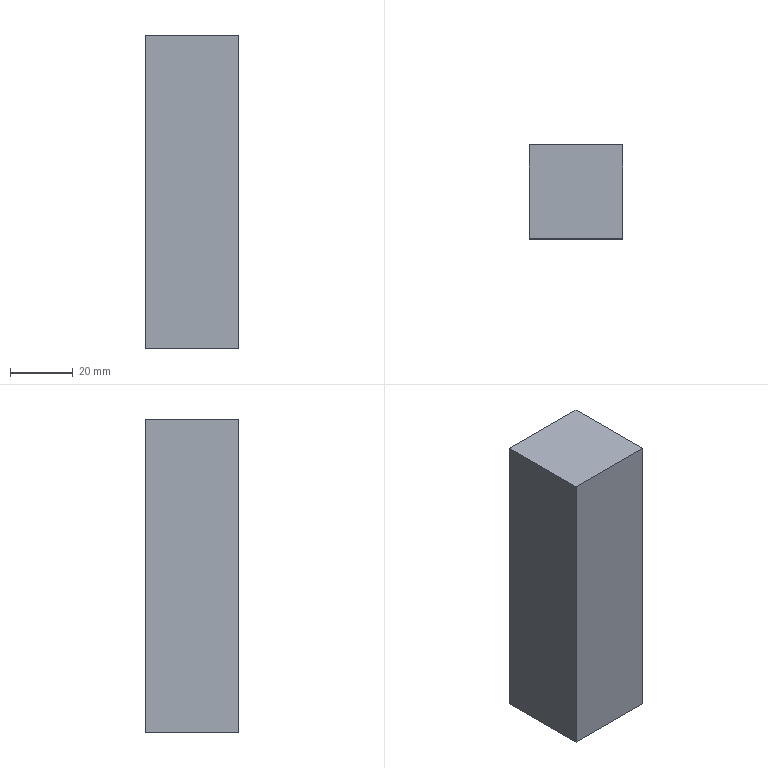Component | NX | FRONT_UP | 1 solid | 6 faces | box 30 x 30 x 100 mm | volume 90000 mm3 | plane 6
STEP:
#1=CARTESIAN_POINT('',(0.,0.,0.));
#2=DIRECTION('',(0.,0.,1.));
#3=DIRECTION('',(1.,0.,0.));
#4=AXIS2_PLACEMENT_3D('',#1,#2,#3);
#5=CARTESIAN_POINT('',(422.662,-30.,80.));
#6=VERTEX_POINT('',#5);
#7=CARTESIAN_POINT('',(422.662,-30.,-20.));
#8=VERTEX_POINT('',#7);
#9=CARTESIAN_POINT('',(422.662,-30.,80.));
#10=DIRECTION('',(0.,0.,-1.));
#11=VECTOR('',#10,1.);
#12=LINE('',#9,#11);
#13=CARTESIAN_POINT('',(422.662,-60.,80.));
#14=DIRECTION('',(1.,0.,0.));
#15=DIRECTION('',(0.,0.,-1.));
#16=AXIS2_PLACEMENT_3D('',#13,#14,#15);
#17=PLANE('',#16);
#18=CARTESIAN_POINT('',(0.,30.));
#19=DIRECTION('',(1.,0.));
#20=VECTOR('',#19,1.);
#21=LINE('',#18,#20);
#22=(GEOMETRIC_REPRESENTATION_CONTEXT(2)PARAMETRIC_REPRESENTATION_CONTEXT()REPRESENTATION_CONTEXT('',''));
#23=DEFINITIONAL_REPRESENTATION('',(#21),#22);
#24=PCURVE('',#17,#23);
#25=CARTESIAN_POINT('',(422.662,-30.,-20.));
#26=DIRECTION('',(0.,-1.,0.));
#27=DIRECTION('',(0.,0.,-1.));
#28=AXIS2_PLACEMENT_3D('',#25,#26,#27);
#29=PLANE('',#28);
#30=CARTESIAN_POINT('',(-100.,0.));
#31=DIRECTION('',(1.,0.));
#32=VECTOR('',#31,1.);
#33=LINE('',#30,#32);
#34=(GEOMETRIC_REPRESENTATION_CONTEXT(2)PARAMETRIC_REPRESENTATION_CONTEXT()REPRESENTATION_CONTEXT('',''));
#35=DEFINITIONAL_REPRESENTATION('',(#33),#34);
#36=PCURVE('',#29,#35);
#37=SURFACE_CURVE('',#12,(#24,#36),.PCURVE_S1.);
#38=EDGE_CURVE('',#6,#8,#37,.T.);
#39=ORIENTED_EDGE('',*,*,#38,.T.);
#40=CARTESIAN_POINT('',(422.662,-60.,-20.));
#41=VERTEX_POINT('',#40);
#42=CARTESIAN_POINT('',(422.662,-60.,-20.));
#43=DIRECTION('',(0.,1.,0.));
#44=VECTOR('',#43,1.);
#45=LINE('',#42,#44);
#46=CARTESIAN_POINT('',(100.,0.));
#47=DIRECTION('',(0.,1.));
#48=VECTOR('',#47,1.);
#49=LINE('',#46,#48);
#50=(GEOMETRIC_REPRESENTATION_CONTEXT(2)PARAMETRIC_REPRESENTATION_CONTEXT()REPRESENTATION_CONTEXT('',''));
#51=DEFINITIONAL_REPRESENTATION('',(#49),#50);
#52=PCURVE('',#17,#51);
#53=CARTESIAN_POINT('',(422.662,-60.,-20.));
#54=DIRECTION('',(0.,0.,1.));
#55=DIRECTION('',(1.,0.,0.));
#56=AXIS2_PLACEMENT_3D('',#53,#54,#55);
#57=PLANE('',#56);
#58=CARTESIAN_POINT('',(0.,0.));
#59=DIRECTION('',(0.,1.));
#60=VECTOR('',#59,1.);
#61=LINE('',#58,#60);
#62=(GEOMETRIC_REPRESENTATION_CONTEXT(2)PARAMETRIC_REPRESENTATION_CONTEXT()REPRESENTATION_CONTEXT('',''));
#63=DEFINITIONAL_REPRESENTATION('',(#61),#62);
#64=PCURVE('',#57,#63);
#65=SURFACE_CURVE('',#45,(#52,#64),.PCURVE_S1.);
#66=EDGE_CURVE('',#41,#8,#65,.T.);
#67=ORIENTED_EDGE('',*,*,#66,.F.);
#68=CARTESIAN_POINT('',(422.662,-60.,80.));
#69=VERTEX_POINT('',#68);
#70=CARTESIAN_POINT('',(422.662,-60.,80.));
#71=DIRECTION('',(0.,0.,-1.));
#72=VECTOR('',#71,1.);
#73=LINE('',#70,#72);
#74=CARTESIAN_POINT('',(0.,0.));
#75=DIRECTION('',(1.,0.));
#76=VECTOR('',#75,1.);
#77=LINE('',#74,#76);
#78=(GEOMETRIC_REPRESENTATION_CONTEXT(2)PARAMETRIC_REPRESENTATION_CONTEXT()REPRESENTATION_CONTEXT('',''));
#79=DEFINITIONAL_REPRESENTATION('',(#77),#78);
#80=PCURVE('',#17,#79);
#81=CARTESIAN_POINT('',(422.662,-60.,-20.));
#82=DIRECTION('',(0.,-1.,0.));
#83=DIRECTION('',(0.,0.,-1.));
#84=AXIS2_PLACEMENT_3D('',#81,#82,#83);
#85=PLANE('',#84);
#86=CARTESIAN_POINT('',(-100.,0.));
#87=DIRECTION('',(1.,0.));
#88=VECTOR('',#87,1.);
#89=LINE('',#86,#88);
#90=(GEOMETRIC_REPRESENTATION_CONTEXT(2)PARAMETRIC_REPRESENTATION_CONTEXT()REPRESENTATION_CONTEXT('',''));
#91=DEFINITIONAL_REPRESENTATION('',(#89),#90);
#92=PCURVE('',#85,#91);
#93=SURFACE_CURVE('',#73,(#80,#92),.PCURVE_S1.);
#94=EDGE_CURVE('',#69,#41,#93,.T.);
#95=ORIENTED_EDGE('',*,*,#94,.F.);
#96=CARTESIAN_POINT('',(422.662,-60.,80.));
#97=DIRECTION('',(0.,1.,0.));
#98=VECTOR('',#97,1.);
#99=LINE('',#96,#98);
#100=CARTESIAN_POINT('',(0.,0.));
#101=DIRECTION('',(0.,1.));
#102=VECTOR('',#101,1.);
#103=LINE('',#100,#102);
#104=(GEOMETRIC_REPRESENTATION_CONTEXT(2)PARAMETRIC_REPRESENTATION_CONTEXT()REPRESENTATION_CONTEXT('',''));
#105=DEFINITIONAL_REPRESENTATION('',(#103),#104);
#106=PCURVE('',#17,#105);
#107=CARTESIAN_POINT('',(452.662,-60.,80.));
#108=DIRECTION('',(-0.,0.,-1.));
#109=DIRECTION('',(-1.,0.,0.));
#110=AXIS2_PLACEMENT_3D('',#107,#108,#109);
#111=PLANE('',#110);
#112=CARTESIAN_POINT('',(30.,0.));
#113=DIRECTION('',(0.,1.));
#114=VECTOR('',#113,1.);
#115=LINE('',#112,#114);
#116=(GEOMETRIC_REPRESENTATION_CONTEXT(2)PARAMETRIC_REPRESENTATION_CONTEXT()REPRESENTATION_CONTEXT('',''));
#117=DEFINITIONAL_REPRESENTATION('',(#115),#116);
#118=PCURVE('',#111,#117);
#119=SURFACE_CURVE('',#99,(#106,#118),.PCURVE_S1.);
#120=EDGE_CURVE('',#69,#6,#119,.T.);
#121=ORIENTED_EDGE('',*,*,#120,.T.);
#122=EDGE_LOOP('',(#39,#67,#95,#121));
#123=FACE_BOUND('',#122,.T.);
#124=ADVANCED_FACE('',(#123),#17,.F.);
#125=CARTESIAN_POINT('',(452.662,-30.,-20.));
#126=VERTEX_POINT('',#125);
#127=CARTESIAN_POINT('',(422.662,-30.,-20.));
#128=DIRECTION('',(1.,0.,0.));
#129=VECTOR('',#128,1.);
#130=LINE('',#127,#129);
#131=CARTESIAN_POINT('',(0.,30.));
#132=DIRECTION('',(1.,0.));
#133=VECTOR('',#132,1.);
#134=LINE('',#131,#133);
#135=(GEOMETRIC_REPRESENTATION_CONTEXT(2)PARAMETRIC_REPRESENTATION_CONTEXT()REPRESENTATION_CONTEXT('',''));
#136=DEFINITIONAL_REPRESENTATION('',(#134),#135);
#137=PCURVE('',#57,#136);
#138=CARTESIAN_POINT('',(0.,0.));
#139=DIRECTION('',(0.,1.));
#140=VECTOR('',#139,1.);
#141=LINE('',#138,#140);
#142=(GEOMETRIC_REPRESENTATION_CONTEXT(2)PARAMETRIC_REPRESENTATION_CONTEXT()REPRESENTATION_CONTEXT('',''));
#143=DEFINITIONAL_REPRESENTATION('',(#141),#142);
#144=PCURVE('',#29,#143);
#145=SURFACE_CURVE('',#130,(#137,#144),.PCURVE_S1.);
#146=EDGE_CURVE('',#8,#126,#145,.T.);
#147=ORIENTED_EDGE('',*,*,#146,.T.);
#148=CARTESIAN_POINT('',(452.662,-60.,-20.));
#149=VERTEX_POINT('',#148);
#150=CARTESIAN_POINT('',(452.662,-60.,-20.));
#151=DIRECTION('',(0.,1.,0.));
#152=VECTOR('',#151,1.);
#153=LINE('',#150,#152);
#154=CARTESIAN_POINT('',(30.,0.));
#155=DIRECTION('',(0.,1.));
#156=VECTOR('',#155,1.);
#157=LINE('',#154,#156);
#158=(GEOMETRIC_REPRESENTATION_CONTEXT(2)PARAMETRIC_REPRESENTATION_CONTEXT()REPRESENTATION_CONTEXT('',''));
#159=DEFINITIONAL_REPRESENTATION('',(#157),#158);
#160=PCURVE('',#57,#159);
#161=CARTESIAN_POINT('',(452.662,-60.,-20.));
#162=DIRECTION('',(-1.,0.,-0.));
#163=DIRECTION('',(-0.,0.,1.));
#164=AXIS2_PLACEMENT_3D('',#161,#162,#163);
#165=PLANE('',#164);
#166=CARTESIAN_POINT('',(0.,0.));
#167=DIRECTION('',(0.,1.));
#168=VECTOR('',#167,1.);
#169=LINE('',#166,#168);
#170=(GEOMETRIC_REPRESENTATION_CONTEXT(2)PARAMETRIC_REPRESENTATION_CONTEXT()REPRESENTATION_CONTEXT('',''));
#171=DEFINITIONAL_REPRESENTATION('',(#169),#170);
#172=PCURVE('',#165,#171);
#173=SURFACE_CURVE('',#153,(#160,#172),.PCURVE_S1.);
#174=EDGE_CURVE('',#149,#126,#173,.T.);
#175=ORIENTED_EDGE('',*,*,#174,.F.);
#176=CARTESIAN_POINT('',(422.662,-60.,-20.));
#177=DIRECTION('',(1.,0.,0.));
#178=VECTOR('',#177,1.);
#179=LINE('',#176,#178);
#180=CARTESIAN_POINT('',(0.,0.));
#181=DIRECTION('',(1.,0.));
#182=VECTOR('',#181,1.);
#183=LINE('',#180,#182);
#184=(GEOMETRIC_REPRESENTATION_CONTEXT(2)PARAMETRIC_REPRESENTATION_CONTEXT()REPRESENTATION_CONTEXT('',''));
#185=DEFINITIONAL_REPRESENTATION('',(#183),#184);
#186=PCURVE('',#57,#185);
#187=CARTESIAN_POINT('',(0.,0.));
#188=DIRECTION('',(0.,1.));
#189=VECTOR('',#188,1.);
#190=LINE('',#187,#189);
#191=(GEOMETRIC_REPRESENTATION_CONTEXT(2)PARAMETRIC_REPRESENTATION_CONTEXT()REPRESENTATION_CONTEXT('',''));
#192=DEFINITIONAL_REPRESENTATION('',(#190),#191);
#193=PCURVE('',#85,#192);
#194=SURFACE_CURVE('',#179,(#186,#193),.PCURVE_S1.);
#195=EDGE_CURVE('',#41,#149,#194,.T.);
#196=ORIENTED_EDGE('',*,*,#195,.F.);
#197=ORIENTED_EDGE('',*,*,#66,.T.);
#198=EDGE_LOOP('',(#147,#175,#196,#197));
#199=FACE_BOUND('',#198,.T.);
#200=ADVANCED_FACE('',(#199),#57,.F.);
#201=CARTESIAN_POINT('',(452.662,-30.,80.));
#202=VERTEX_POINT('',#201);
#203=CARTESIAN_POINT('',(452.662,-30.,-20.));
#204=DIRECTION('',(-0.,0.,1.));
#205=VECTOR('',#204,1.);
#206=LINE('',#203,#205);
#207=CARTESIAN_POINT('',(0.,30.));
#208=DIRECTION('',(1.,0.));
#209=VECTOR('',#208,1.);
#210=LINE('',#207,#209);
#211=(GEOMETRIC_REPRESENTATION_CONTEXT(2)PARAMETRIC_REPRESENTATION_CONTEXT()REPRESENTATION_CONTEXT('',''));
#212=DEFINITIONAL_REPRESENTATION('',(#210),#211);
#213=PCURVE('',#165,#212);
#214=CARTESIAN_POINT('',(0.,30.));
#215=DIRECTION('',(-1.,-0.));
#216=VECTOR('',#215,1.);
#217=LINE('',#214,#216);
#218=(GEOMETRIC_REPRESENTATION_CONTEXT(2)PARAMETRIC_REPRESENTATION_CONTEXT()REPRESENTATION_CONTEXT('',''));
#219=DEFINITIONAL_REPRESENTATION('',(#217),#218);
#220=PCURVE('',#29,#219);
#221=SURFACE_CURVE('',#206,(#213,#220),.PCURVE_S1.);
#222=EDGE_CURVE('',#126,#202,#221,.T.);
#223=ORIENTED_EDGE('',*,*,#222,.T.);
#224=CARTESIAN_POINT('',(452.662,-60.,80.));
#225=VERTEX_POINT('',#224);
#226=CARTESIAN_POINT('',(452.662,-60.,80.));
#227=DIRECTION('',(0.,1.,0.));
#228=VECTOR('',#227,1.);
#229=LINE('',#226,#228);
#230=CARTESIAN_POINT('',(100.,0.));
#231=DIRECTION('',(0.,1.));
#232=VECTOR('',#231,1.);
#233=LINE('',#230,#232);
#234=(GEOMETRIC_REPRESENTATION_CONTEXT(2)PARAMETRIC_REPRESENTATION_CONTEXT()REPRESENTATION_CONTEXT('',''));
#235=DEFINITIONAL_REPRESENTATION('',(#233),#234);
#236=PCURVE('',#165,#235);
#237=CARTESIAN_POINT('',(0.,0.));
#238=DIRECTION('',(0.,1.));
#239=VECTOR('',#238,1.);
#240=LINE('',#237,#239);
#241=(GEOMETRIC_REPRESENTATION_CONTEXT(2)PARAMETRIC_REPRESENTATION_CONTEXT()REPRESENTATION_CONTEXT('',''));
#242=DEFINITIONAL_REPRESENTATION('',(#240),#241);
#243=PCURVE('',#111,#242);
#244=SURFACE_CURVE('',#229,(#236,#243),.PCURVE_S1.);
#245=EDGE_CURVE('',#225,#202,#244,.T.);
#246=ORIENTED_EDGE('',*,*,#245,.F.);
#247=CARTESIAN_POINT('',(452.662,-60.,-20.));
#248=DIRECTION('',(-0.,0.,1.));
#249=VECTOR('',#248,1.);
#250=LINE('',#247,#249);
#251=CARTESIAN_POINT('',(0.,0.));
#252=DIRECTION('',(1.,0.));
#253=VECTOR('',#252,1.);
#254=LINE('',#251,#253);
#255=(GEOMETRIC_REPRESENTATION_CONTEXT(2)PARAMETRIC_REPRESENTATION_CONTEXT()REPRESENTATION_CONTEXT('',''));
#256=DEFINITIONAL_REPRESENTATION('',(#254),#255);
#257=PCURVE('',#165,#256);
#258=CARTESIAN_POINT('',(0.,30.));
#259=DIRECTION('',(-1.,-0.));
#260=VECTOR('',#259,1.);
#261=LINE('',#258,#260);
#262=(GEOMETRIC_REPRESENTATION_CONTEXT(2)PARAMETRIC_REPRESENTATION_CONTEXT()REPRESENTATION_CONTEXT('',''));
#263=DEFINITIONAL_REPRESENTATION('',(#261),#262);
#264=PCURVE('',#85,#263);
#265=SURFACE_CURVE('',#250,(#257,#264),.PCURVE_S1.);
#266=EDGE_CURVE('',#149,#225,#265,.T.);
#267=ORIENTED_EDGE('',*,*,#266,.F.);
#268=ORIENTED_EDGE('',*,*,#174,.T.);
#269=EDGE_LOOP('',(#223,#246,#267,#268));
#270=FACE_BOUND('',#269,.T.);
#271=ADVANCED_FACE('',(#270),#165,.F.);
#272=CARTESIAN_POINT('',(452.662,-30.,80.));
#273=DIRECTION('',(-1.,0.,0.));
#274=VECTOR('',#273,1.);
#275=LINE('',#272,#274);
#276=CARTESIAN_POINT('',(0.,30.));
#277=DIRECTION('',(1.,0.));
#278=VECTOR('',#277,1.);
#279=LINE('',#276,#278);
#280=(GEOMETRIC_REPRESENTATION_CONTEXT(2)PARAMETRIC_REPRESENTATION_CONTEXT()REPRESENTATION_CONTEXT('',''));
#281=DEFINITIONAL_REPRESENTATION('',(#279),#280);
#282=PCURVE('',#111,#281);
#283=CARTESIAN_POINT('',(-100.,30.));
#284=DIRECTION('',(-0.,-1.));
#285=VECTOR('',#284,1.);
#286=LINE('',#283,#285);
#287=(GEOMETRIC_REPRESENTATION_CONTEXT(2)PARAMETRIC_REPRESENTATION_CONTEXT()REPRESENTATION_CONTEXT('',''));
#288=DEFINITIONAL_REPRESENTATION('',(#286),#287);
#289=PCURVE('',#29,#288);
#290=SURFACE_CURVE('',#275,(#282,#289),.PCURVE_S1.);
#291=EDGE_CURVE('',#202,#6,#290,.T.);
#292=ORIENTED_EDGE('',*,*,#291,.T.);
#293=ORIENTED_EDGE('',*,*,#120,.F.);
#294=CARTESIAN_POINT('',(452.662,-60.,80.));
#295=DIRECTION('',(-1.,0.,0.));
#296=VECTOR('',#295,1.);
#297=LINE('',#294,#296);
#298=CARTESIAN_POINT('',(0.,0.));
#299=DIRECTION('',(1.,0.));
#300=VECTOR('',#299,1.);
#301=LINE('',#298,#300);
#302=(GEOMETRIC_REPRESENTATION_CONTEXT(2)PARAMETRIC_REPRESENTATION_CONTEXT()REPRESENTATION_CONTEXT('',''));
#303=DEFINITIONAL_REPRESENTATION('',(#301),#302);
#304=PCURVE('',#111,#303);
#305=CARTESIAN_POINT('',(-100.,30.));
#306=DIRECTION('',(-0.,-1.));
#307=VECTOR('',#306,1.);
#308=LINE('',#305,#307);
#309=(GEOMETRIC_REPRESENTATION_CONTEXT(2)PARAMETRIC_REPRESENTATION_CONTEXT()REPRESENTATION_CONTEXT('',''));
#310=DEFINITIONAL_REPRESENTATION('',(#308),#309);
#311=PCURVE('',#85,#310);
#312=SURFACE_CURVE('',#297,(#304,#311),.PCURVE_S1.);
#313=EDGE_CURVE('',#225,#69,#312,.T.);
#314=ORIENTED_EDGE('',*,*,#313,.F.);
#315=ORIENTED_EDGE('',*,*,#245,.T.);
#316=EDGE_LOOP('',(#292,#293,#314,#315));
#317=FACE_BOUND('',#316,.T.);
#318=ADVANCED_FACE('',(#317),#111,.F.);
#319=ORIENTED_EDGE('',*,*,#94,.T.);
#320=ORIENTED_EDGE('',*,*,#195,.T.);
#321=ORIENTED_EDGE('',*,*,#266,.T.);
#322=ORIENTED_EDGE('',*,*,#313,.T.);
#323=EDGE_LOOP('',(#319,#320,#321,#322));
#324=FACE_BOUND('',#323,.T.);
#325=ADVANCED_FACE('',(#324),#85,.T.);
#326=ORIENTED_EDGE('',*,*,#38,.F.);
#327=ORIENTED_EDGE('',*,*,#291,.F.);
#328=ORIENTED_EDGE('',*,*,#222,.F.);
#329=ORIENTED_EDGE('',*,*,#146,.F.);
#330=EDGE_LOOP('',(#326,#327,#328,#329));
#331=FACE_BOUND('',#330,.T.);
#332=ADVANCED_FACE('',(#331),#29,.F.);
#333=CLOSED_SHELL('',(#124,#200,#271,#318,#325,#332));
#334=MANIFOLD_SOLID_BREP('',#333);
#335=(LENGTH_UNIT()NAMED_UNIT(*)SI_UNIT(.MILLI.,.METRE.));
#336=UNCERTAINTY_MEASURE_WITH_UNIT(LENGTH_MEASURE(0.0000001),#335,'','');
#337=(NAMED_UNIT(*)PLANE_ANGLE_UNIT()SI_UNIT($,.RADIAN.));
#338=(NAMED_UNIT(*)SI_UNIT($,.STERADIAN.)SOLID_ANGLE_UNIT());
#339=(GEOMETRIC_REPRESENTATION_CONTEXT(3)GLOBAL_UNCERTAINTY_ASSIGNED_CONTEXT((#336))GLOBAL_UNIT_ASSIGNED_CONTEXT((#335,#337,#338))REPRESENTATION_CONTEXT('',''));
#340=ADVANCED_BREP_SHAPE_REPRESENTATION('',(#4,#334),#339);